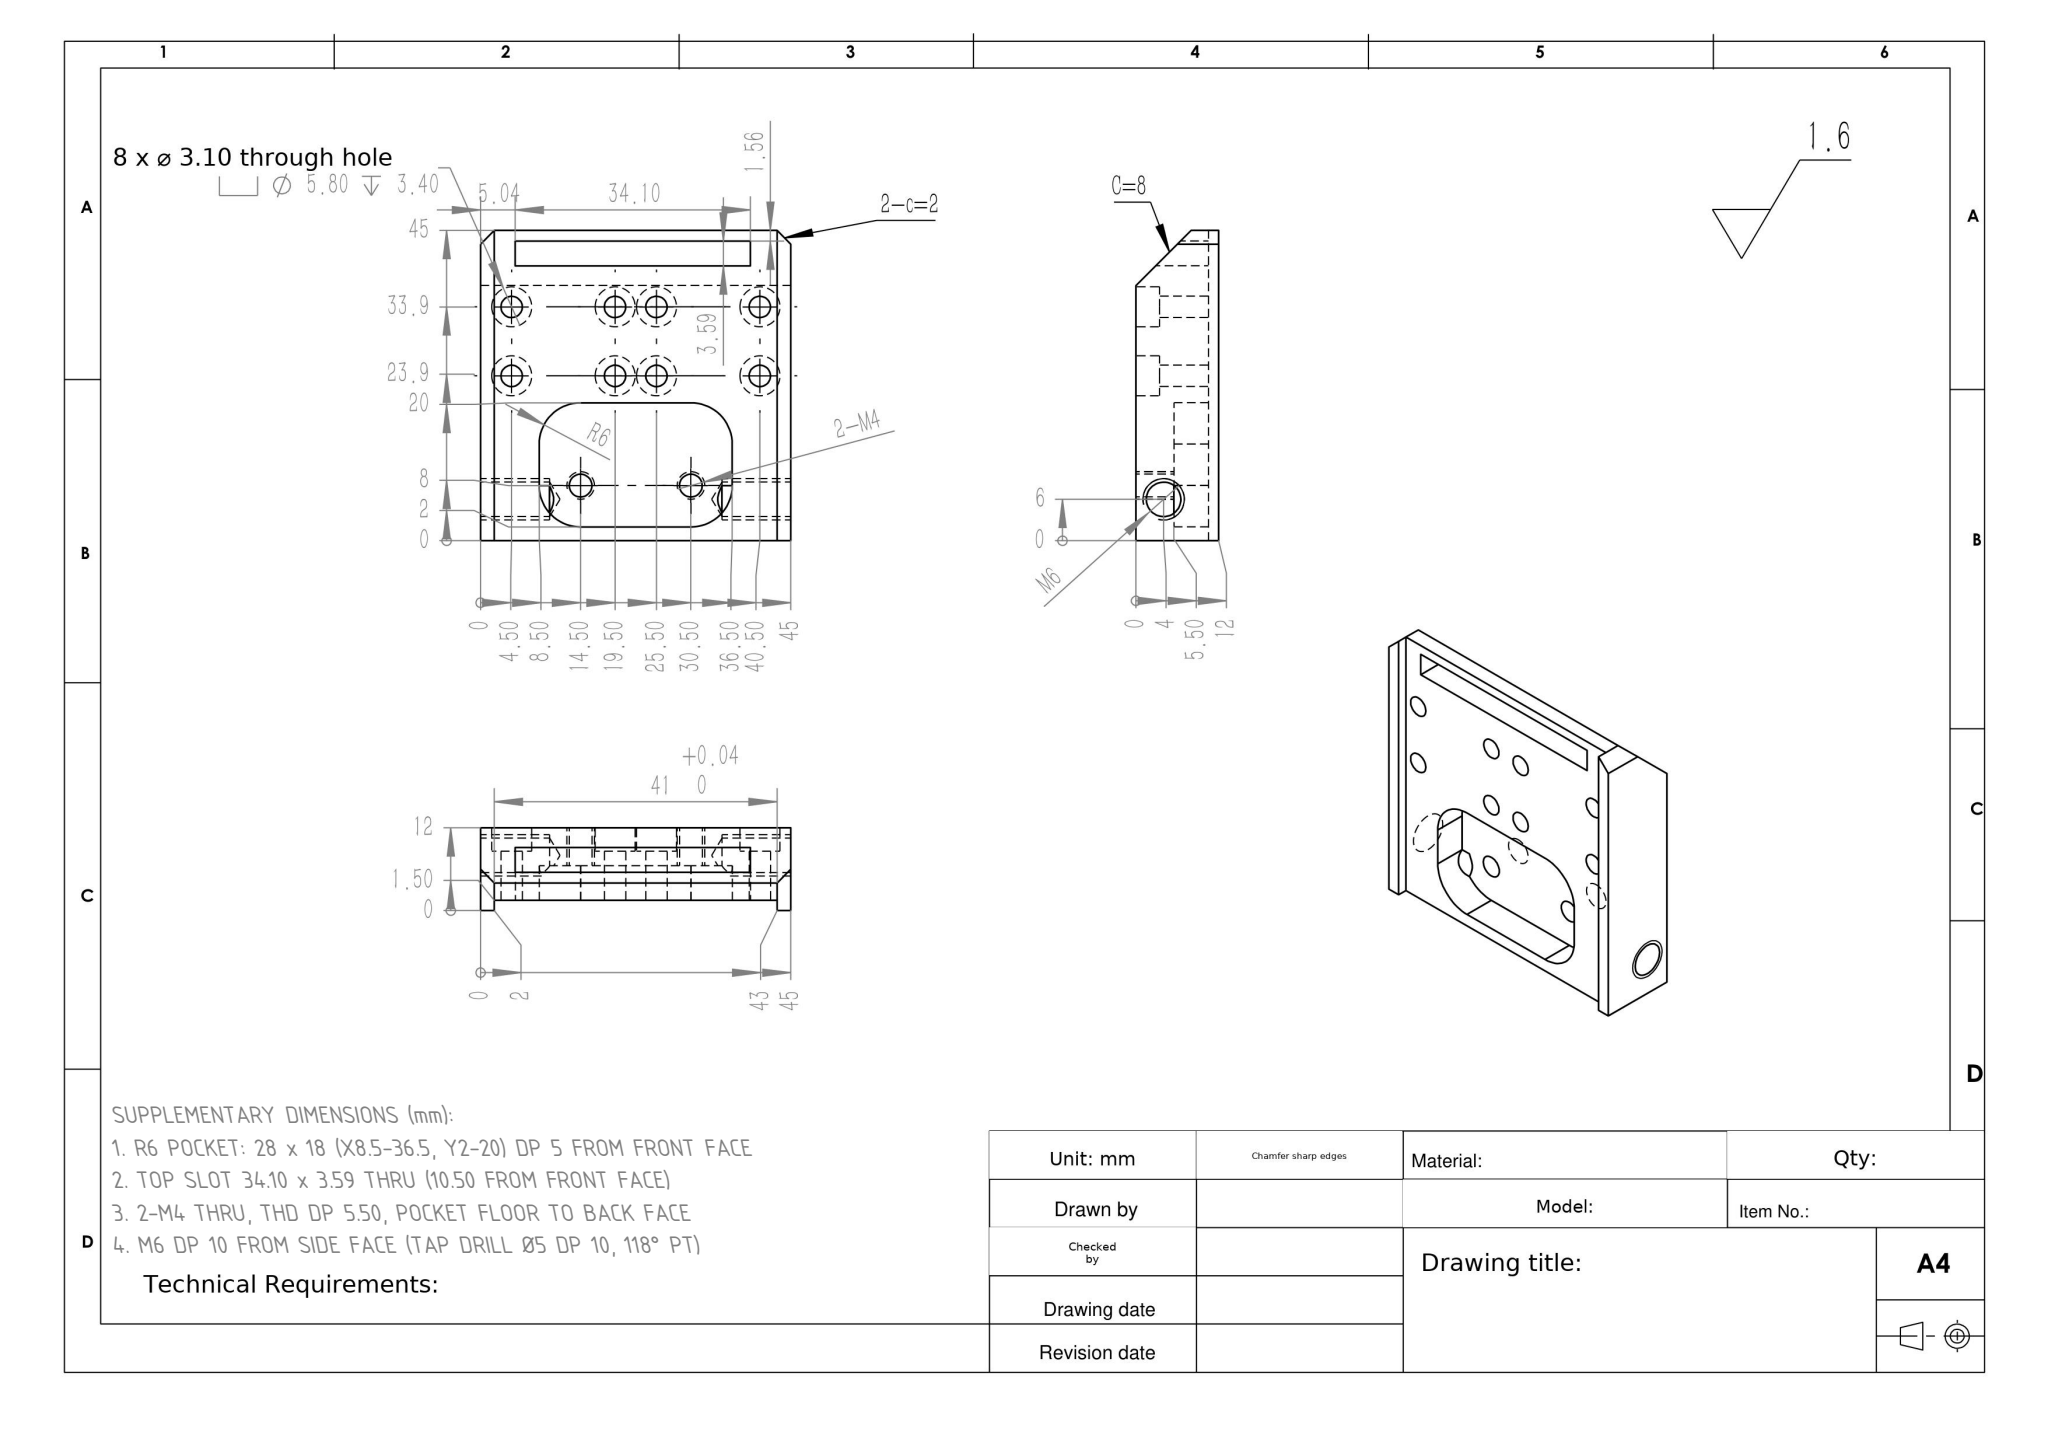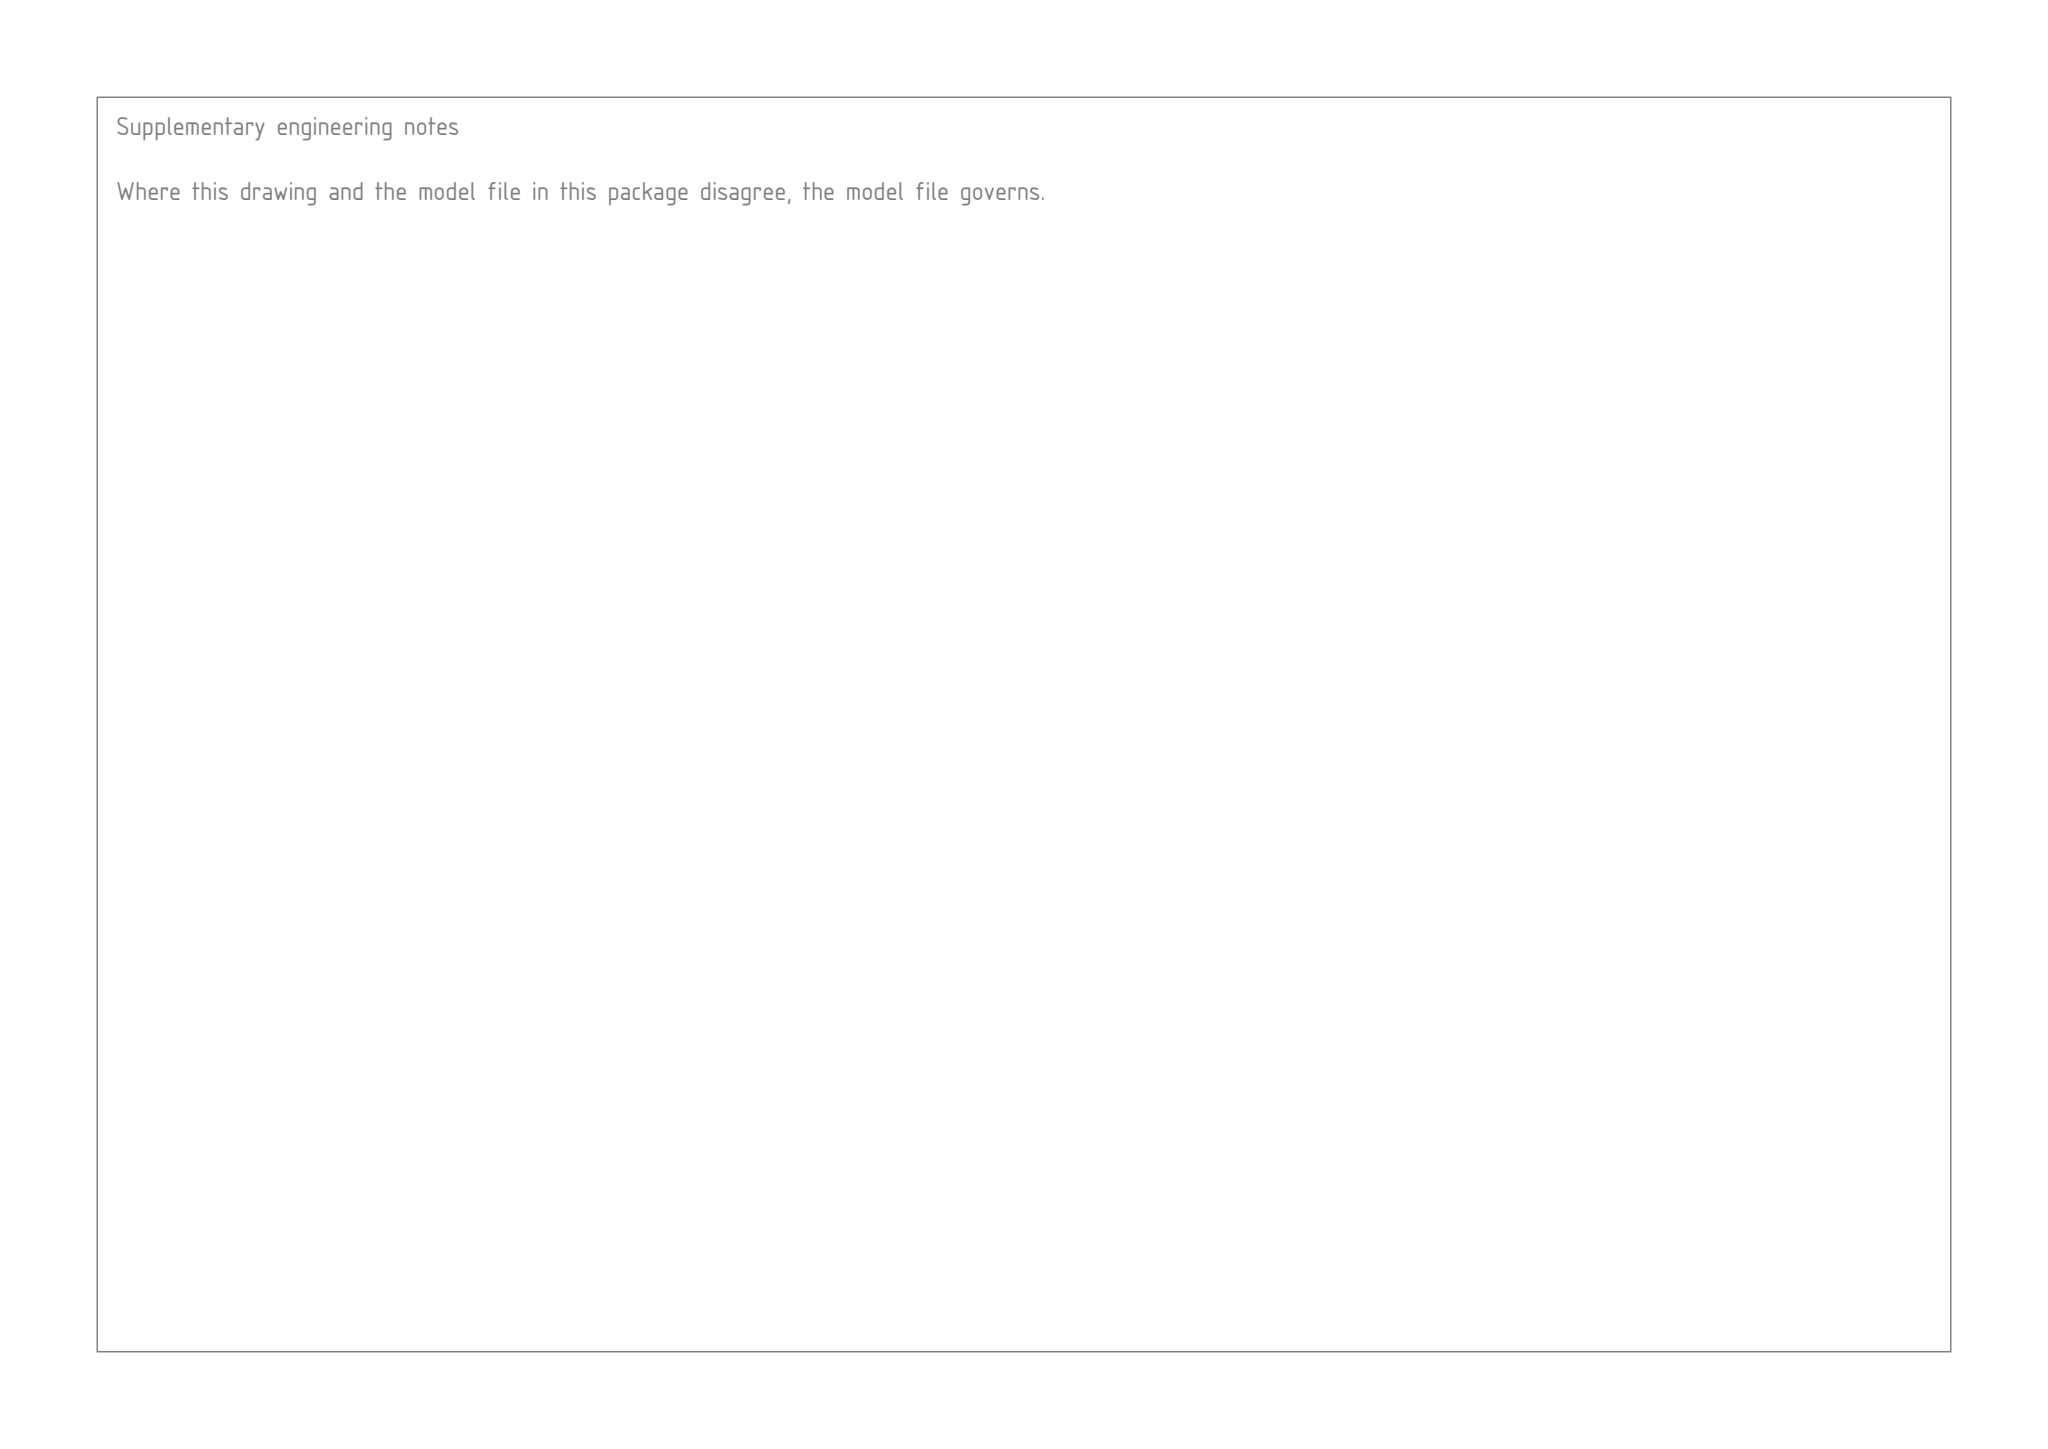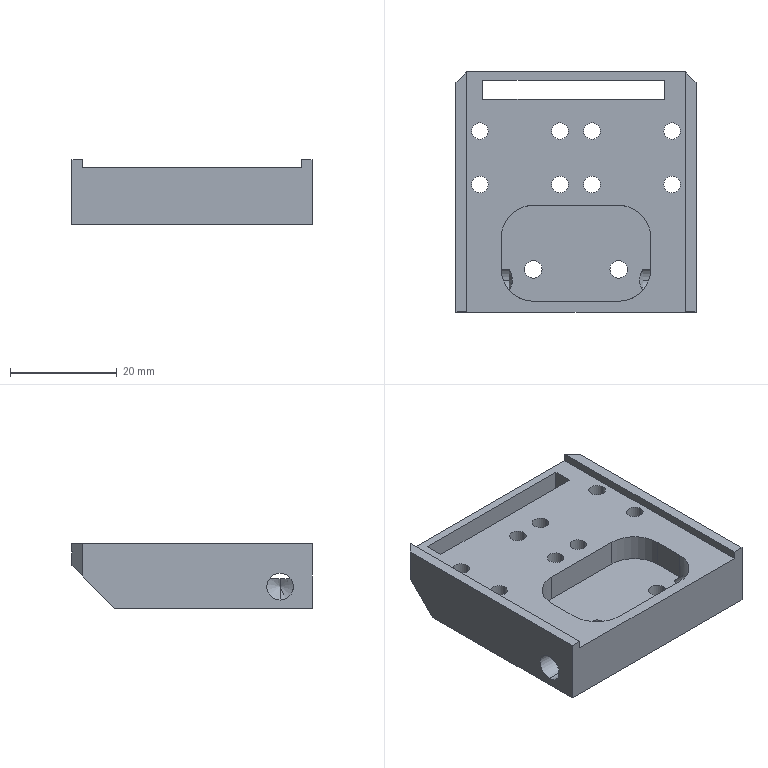Part | SolidWorks | mm | 1 solid | 78 faces | box 45 x 45 x 12 mm | volume 15344 mm3 | cylinder 44 | plane 30 | cone 4 | commonest cylinder face diameters 5.8 x16 3.1 x16 5 x4 3.3 x4 12 x4
build123d program:
from build123d import *

# Parameters (mm, degrees)
SKETCH1_W                                            = 45
SKETCH1_H                                            = 45
BOSS_EXTRUDE1_DEPTH                                  = 12
SKETCH3_W                                            = 41
SKETCH3_H                                            = 45
CUT_EXTRUDE2_DEPTH                                   = 1.5
M4_TAPPED_HOLE1_D                                    = 3.3
M4_TAPPED_HOLE1_DEPTH                                = 11.5
M4_TAPPED_HOLE1_TIP                                  = 0.9914
CHAMFER1_SIZE                                        = 2
HOLE_SIZE_ACCORDING_TO_THE_TYPE_OF_HEX_S_D           = 3.1
HOLE_SIZE_ACCORDING_TO_THE_TYPE_OF_HEX_S_CBORE_D     = 5.8
HOLE_SIZE_ACCORDING_TO_THE_TYPE_OF_HEX_S_CBORE_DEPTH = 3.4
CHAMFER2_SIZE                                        = 8
CUT_EXTRUDE3_DEPTH                                   = 5
SKETCH12_W                                           = 34.099
SKETCH12_H                                           = 3.594
CUT_EXTRUDE4_DEPTH                                   = 10


with BuildPart() as part:
    # Sketch1 → Boss-Extrude1 (new body)
    with BuildSketch(Plane.XY):
        with Locations((-22.5, 22.5)):
            Rectangle(SKETCH1_W, SKETCH1_H)
    extrude(amount=BOSS_EXTRUDE1_DEPTH)

    # Sketch3 → Cut-Extrude2 (cut)
    with BuildSketch(Plane.XY.offset(12)):
        with Locations((-22.5, 22.5)):
            Rectangle(SKETCH3_W, SKETCH3_H)
    extrude(amount=-CUT_EXTRUDE2_DEPTH, mode=Mode.SUBTRACT)

    # Sketch4 → M6 Tapped Hole1 (revolve, cut)
    with BuildSketch(Plane(origin=(-45, 6, 4), x_dir=(0, 0, 1), z_dir=(0, 1, 0))):
        Polygon((0, 0), (0, 11.502), (2.5, 10), (2.5, 0), align=None)
    m6_tapped_hole1 = revolve(axis=Axis((-51.35, 6, 4), (1, 0, 0)), mode=Mode.SUBTRACT)

    # M4 Tapped Hole1
    with Locations(Plane(origin=(0, 0, 0), x_dir=(-1, 0, 0), z_dir=(0, 0, -1))):
        with Locations((14.5, 8), (30.5, 8)):
            Hole(M4_TAPPED_HOLE1_D / 2, depth=M4_TAPPED_HOLE1_DEPTH)
            with Locations((0, 0, -(M4_TAPPED_HOLE1_DEPTH + M4_TAPPED_HOLE1_TIP / 2))):  # 118° drill point
                Cone(0, M4_TAPPED_HOLE1_D / 2, M4_TAPPED_HOLE1_TIP, mode=Mode.SUBTRACT)

    # Chamfer1
    chamfer1_edges = [part.edges().sort_by_distance(p)[0] for p in [
        (-45, 45, 6),
        (0, 45, 6),
    ]]
    chamfer(chamfer1_edges, length=CHAMFER1_SIZE)

    # Hole Size according to the type of hex s (through all)
    with Locations(Plane(origin=(0, 0, 0), x_dir=(-1, 0, 0), z_dir=(0, 0, -1))):
        with Locations((19.5, 33.9), (19.5, 23.9), (4.5, 23.9), (4.5, 33.9), (40.5, 33.9), (40.5, 23.9), (25.5, 23.9), (25.5, 33.9)):
            CounterBoreHole(HOLE_SIZE_ACCORDING_TO_THE_TYPE_OF_HEX_S_D / 2, HOLE_SIZE_ACCORDING_TO_THE_TYPE_OF_HEX_S_CBORE_D / 2, HOLE_SIZE_ACCORDING_TO_THE_TYPE_OF_HEX_S_CBORE_DEPTH)

    # Chamfer2
    chamfer2_edges = [part.edges().sort_by_distance(p)[0] for p in [
        (-22.5, 45, 0),
    ]]
    chamfer(chamfer2_edges, length=CHAMFER2_SIZE)

    # Sketch11 → Cut-Extrude3 (cut)
    with BuildSketch(Plane.XY.offset(10.5)):
        with BuildLine():
            Line((-30.5, 2), (-14.5, 2))
            ThreePointArc((-14.5, 2), (-10.257, 3.757), (-8.5, 8))
            Line((-8.5, 8), (-8.5, 14))
            ThreePointArc((-8.5, 14), (-10.257, 18.243), (-14.5, 20))
            Line((-14.5, 20), (-30.5, 20))
            ThreePointArc((-30.5, 20), (-34.743, 18.243), (-36.5, 14))
            Line((-36.5, 14), (-36.5, 8))
            ThreePointArc((-36.5, 8), (-34.743, 3.757), (-30.5, 2))
        make_face()
    extrude(amount=-CUT_EXTRUDE3_DEPTH, mode=Mode.SUBTRACT)

    # Mirror1: M6 Tapped Hole1 across plane
    add(m6_tapped_hole1.mirror(Plane.ZY.offset(22.5)), mode=Mode.SUBTRACT)

    # Sketch12 → Cut-Extrude4 (cut)
    with BuildSketch(Plane.XY.offset(10.5)):
        with Locations((-22.915, 41.646)):
            Rectangle(SKETCH12_W, SKETCH12_H)
    extrude(amount=-CUT_EXTRUDE4_DEPTH, mode=Mode.SUBTRACT)


solid = part.part